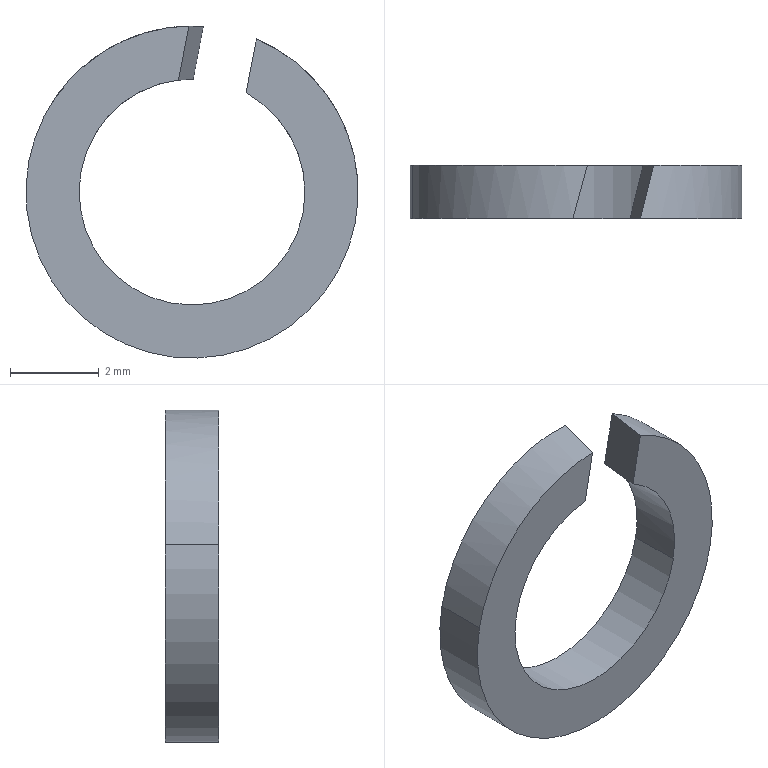Component | SolidWorks | SpringWasher_5-2 | 1 solid | 10 faces | box 7.5 x 1.2 x 7.5 mm | volume 26 mm3 | cylinder 6 | plane 4 | commonest cylinder face diameters 5.1 x3 7.5 x3 | material Plain Carbon Steel
build123d program:
from build123d import *

# Parameters (mm, degrees)
SKETCH1_R           = 3.75
SKETCH1_R_2         = 2.55
BOSS_EXTRUDE1_DEPTH = 1.2
CUT_EXTRUDE1_DEPTH  = 6.437


with BuildPart() as part:
    # Sketch1 → Boss-Extrude1 (new body)
    with BuildSketch(Plane.XY):
        Circle(SKETCH1_R)
        Circle(SKETCH1_R_2, mode=Mode.SUBTRACT)
    extrude(amount=BOSS_EXTRUDE1_DEPTH)

    # Sketch2 → Cut-Extrude1 (cut, through all)
    with BuildSketch(Plane(origin=(0, 0, 0), x_dir=(1, 0, 0), z_dir=(0, 1, 0))):
        Polygon((-0.4549, -1.2), (-0.7765, 0), (0.7765, 0), (1.098, -1.2), align=None)
    extrude(amount=-CUT_EXTRUDE1_DEPTH, mode=Mode.SUBTRACT)


solid = part.part

# Placed as in the assembly
solid = solid.moved(Location((-144.749, -17, 133.251), (-90, 0, 10.863)))
STEP:
#1=CARTESIAN_POINT('',(-5.639,-0.622,5.327));
#2=VERTEX_POINT('',#1);
#3=CARTESIAN_POINT('',(-5.6,-0.622,5.227));
#4=VERTEX_POINT('',#3);
#5=CARTESIAN_POINT('',(-5.699,-0.622,5.246));
#6=DIRECTION('',(-0.,1.,0.));
#7=DIRECTION('',(0.9821,0.,-0.1885));
#8=AXIS2_PLACEMENT_3D('',#5,#6,#7);
#9=CIRCLE('',#8,0.1004);
#10=EDGE_CURVE('',#2,#4,#9,.T.);
#11=ORIENTED_EDGE('',*,*,#10,.T.);
#12=CARTESIAN_POINT('',(-5.6,-0.6693,5.227));
#13=VERTEX_POINT('',#12);
#14=CARTESIAN_POINT('',(-5.6,-0.622,5.227));
#15=DIRECTION('',(0.,-1.,-0.));
#16=VECTOR('',#15,39.37);
#17=LINE('',#14,#16);
#18=EDGE_CURVE('',#4,#13,#17,.T.);
#19=ORIENTED_EDGE('',*,*,#18,.T.);
#20=CARTESIAN_POINT('',(-5.651,-0.6693,5.334));
#21=VERTEX_POINT('',#20);
#22=CARTESIAN_POINT('',(-5.699,-0.6693,5.246));
#23=DIRECTION('',(-0.,1.,0.));
#24=DIRECTION('',(0.9821,0.,-0.1885));
#25=AXIS2_PLACEMENT_3D('',#22,#23,#24);
#26=CIRCLE('',#25,0.1004);
#27=EDGE_CURVE('',#21,#13,#26,.T.);
#28=ORIENTED_EDGE('',*,*,#27,.F.);
#29=CARTESIAN_POINT('',(-5.639,-0.622,5.327));
#30=CARTESIAN_POINT('',(-5.643,-0.6374,5.33));
#31=CARTESIAN_POINT('',(-5.647,-0.6531,5.332));
#32=CARTESIAN_POINT('',(-5.651,-0.6693,5.334));
#33=(BOUNDED_CURVE()B_SPLINE_CURVE(3,(#29,#30,#31,#32),.UNSPECIFIED.,.F.,.F.)B_SPLINE_CURVE_WITH_KNOTS((4,4),(4.267,4.403),.UNSPECIFIED.)CURVE()GEOMETRIC_REPRESENTATION_ITEM()RATIONAL_B_SPLINE_CURVE((1.,0.9985,0.9985,1.))REPRESENTATION_ITEM(''));
#34=EDGE_CURVE('',#2,#21,#33,.T.);
#35=ORIENTED_EDGE('',*,*,#34,.F.);
#36=EDGE_LOOP('',(#11,#19,#28,#35));
#37=FACE_OUTER_BOUND('',#36,.T.);
#38=CARTESIAN_POINT('',(-5.699,-0.622,5.246));
#39=DIRECTION('',(0.,-1.,-0.));
#40=DIRECTION('',(-0.9821,0.,0.1885));
#41=AXIS2_PLACEMENT_3D('',#38,#39,#40);
#42=CYLINDRICAL_SURFACE('',#41,0.1004);
#43=ADVANCED_FACE('',(#37),#42,.F.);
#44=ORIENTED_EDGE('',*,*,#18,.F.);
#45=CARTESIAN_POINT('',(-5.797,-0.622,5.265));
#46=VERTEX_POINT('',#45);
#47=CARTESIAN_POINT('',(-5.699,-0.622,5.246));
#48=DIRECTION('',(-0.,1.,0.));
#49=DIRECTION('',(0.9821,0.,-0.1885));
#50=AXIS2_PLACEMENT_3D('',#47,#48,#49);
#51=CIRCLE('',#50,0.1004);
#52=EDGE_CURVE('',#4,#46,#51,.T.);
#53=ORIENTED_EDGE('',*,*,#52,.T.);
#54=CARTESIAN_POINT('',(-5.797,-0.6693,5.265));
#55=VERTEX_POINT('',#54);
#56=CARTESIAN_POINT('',(-5.797,-0.622,5.265));
#57=DIRECTION('',(0.,-1.,-0.));
#58=VECTOR('',#57,39.37);
#59=LINE('',#56,#58);
#60=EDGE_CURVE('',#46,#55,#59,.T.);
#61=ORIENTED_EDGE('',*,*,#60,.T.);
#62=CARTESIAN_POINT('',(-5.699,-0.6693,5.246));
#63=DIRECTION('',(-0.,1.,0.));
#64=DIRECTION('',(0.9821,0.,-0.1885));
#65=AXIS2_PLACEMENT_3D('',#62,#63,#64);
#66=CIRCLE('',#65,0.1004);
#67=EDGE_CURVE('',#13,#55,#66,.T.);
#68=ORIENTED_EDGE('',*,*,#67,.F.);
#69=EDGE_LOOP('',(#44,#53,#61,#68));
#70=FACE_OUTER_BOUND('',#69,.T.);
#71=CARTESIAN_POINT('',(-5.699,-0.622,5.246));
#72=DIRECTION('',(0.,-1.,-0.));
#73=DIRECTION('',(-0.9821,0.,0.1885));
#74=AXIS2_PLACEMENT_3D('',#71,#72,#73);
#75=CYLINDRICAL_SURFACE('',#74,0.1004);
#76=ADVANCED_FACE('',(#70),#75,.F.);
#77=CARTESIAN_POINT('',(-5.554,-0.622,5.218));
#78=VERTEX_POINT('',#77);
#79=CARTESIAN_POINT('',(-5.844,-0.622,5.274));
#80=VERTEX_POINT('',#79);
#81=CARTESIAN_POINT('',(-5.699,-0.622,5.246));
#82=DIRECTION('',(-0.,1.,0.));
#83=DIRECTION('',(0.9821,0.,-0.1885));
#84=AXIS2_PLACEMENT_3D('',#81,#82,#83);
#85=CIRCLE('',#84,0.1476);
#86=EDGE_CURVE('',#78,#80,#85,.T.);
#87=ORIENTED_EDGE('',*,*,#86,.F.);
#88=CARTESIAN_POINT('',(-5.554,-0.6693,5.218));
#89=VERTEX_POINT('',#88);
#90=CARTESIAN_POINT('',(-5.554,-0.622,5.218));
#91=DIRECTION('',(0.,-1.,-0.));
#92=VECTOR('',#91,39.37);
#93=LINE('',#90,#92);
#94=EDGE_CURVE('',#78,#89,#93,.T.);
#95=ORIENTED_EDGE('',*,*,#94,.T.);
#96=CARTESIAN_POINT('',(-5.844,-0.6693,5.274));
#97=VERTEX_POINT('',#96);
#98=CARTESIAN_POINT('',(-5.699,-0.6693,5.246));
#99=DIRECTION('',(-0.,1.,0.));
#100=DIRECTION('',(0.9821,0.,-0.1885));
#101=AXIS2_PLACEMENT_3D('',#98,#99,#100);
#102=CIRCLE('',#101,0.1476);
#103=EDGE_CURVE('',#89,#97,#102,.T.);
#104=ORIENTED_EDGE('',*,*,#103,.T.);
#105=CARTESIAN_POINT('',(-5.844,-0.622,5.274));
#106=DIRECTION('',(0.,-1.,-0.));
#107=VECTOR('',#106,39.37);
#108=LINE('',#105,#107);
#109=EDGE_CURVE('',#80,#97,#108,.T.);
#110=ORIENTED_EDGE('',*,*,#109,.F.);
#111=EDGE_LOOP('',(#87,#95,#104,#110));
#112=FACE_OUTER_BOUND('',#111,.T.);
#113=CARTESIAN_POINT('',(-5.699,-0.622,5.246));
#114=DIRECTION('',(0.,-1.,-0.));
#115=DIRECTION('',(-0.9821,0.,0.1885));
#116=AXIS2_PLACEMENT_3D('',#113,#114,#115);
#117=CYLINDRICAL_SURFACE('',#116,0.1476);
#118=ADVANCED_FACE('',(#112),#117,.T.);
#119=CARTESIAN_POINT('',(-5.689,-0.622,5.393));
#120=VERTEX_POINT('',#119);
#121=CARTESIAN_POINT('',(-5.699,-0.622,5.246));
#122=DIRECTION('',(-0.,1.,0.));
#123=DIRECTION('',(0.9821,0.,-0.1885));
#124=AXIS2_PLACEMENT_3D('',#121,#122,#123);
#125=CIRCLE('',#124,0.1476);
#126=EDGE_CURVE('',#80,#120,#125,.T.);
#127=ORIENTED_EDGE('',*,*,#126,.F.);
#128=ORIENTED_EDGE('',*,*,#109,.T.);
#129=CARTESIAN_POINT('',(-5.702,-0.6693,5.394));
#130=VERTEX_POINT('',#129);
#131=CARTESIAN_POINT('',(-5.699,-0.6693,5.246));
#132=DIRECTION('',(-0.,1.,0.));
#133=DIRECTION('',(0.9821,0.,-0.1885));
#134=AXIS2_PLACEMENT_3D('',#131,#132,#133);
#135=CIRCLE('',#134,0.1476);
#136=EDGE_CURVE('',#97,#130,#135,.T.);
#137=ORIENTED_EDGE('',*,*,#136,.T.);
#138=CARTESIAN_POINT('',(-5.702,-0.6693,5.394));
#139=CARTESIAN_POINT('',(-5.697,-0.6537,5.394));
#140=CARTESIAN_POINT('',(-5.693,-0.6379,5.394));
#141=CARTESIAN_POINT('',(-5.689,-0.622,5.393));
#142=(BOUNDED_CURVE()B_SPLINE_CURVE(3,(#138,#139,#140,#141),.UNSPECIFIED.,.F.,.T.)B_SPLINE_CURVE_WITH_KNOTS((4,4),(1.362,1.449),.UNSPECIFIED.)CURVE()GEOMETRIC_REPRESENTATION_ITEM()RATIONAL_B_SPLINE_CURVE((1.,0.9994,0.9994,1.))REPRESENTATION_ITEM(''));
#143=EDGE_CURVE('',#130,#120,#142,.T.);
#144=ORIENTED_EDGE('',*,*,#143,.T.);
#145=EDGE_LOOP('',(#127,#128,#137,#144));
#146=FACE_OUTER_BOUND('',#145,.T.);
#147=CARTESIAN_POINT('',(-5.699,-0.622,5.246));
#148=DIRECTION('',(0.,-1.,-0.));
#149=DIRECTION('',(-0.9821,0.,0.1885));
#150=AXIS2_PLACEMENT_3D('',#147,#148,#149);
#151=CYLINDRICAL_SURFACE('',#150,0.1476);
#152=ADVANCED_FACE('',(#146),#151,.T.);
#153=CARTESIAN_POINT('',(-5.698,-0.622,5.347));
#154=VERTEX_POINT('',#153);
#155=CARTESIAN_POINT('',(-5.689,-0.622,5.394));
#156=DIRECTION('',(-0.1885,0.,-0.9821));
#157=VECTOR('',#156,39.37);
#158=LINE('',#155,#157);
#159=EDGE_CURVE('',#120,#154,#158,.T.);
#160=ORIENTED_EDGE('',*,*,#159,.T.);
#161=CARTESIAN_POINT('',(-5.699,-0.622,5.246));
#162=DIRECTION('',(-0.,1.,0.));
#163=DIRECTION('',(0.9821,0.,-0.1885));
#164=AXIS2_PLACEMENT_3D('',#161,#162,#163);
#165=CIRCLE('',#164,0.1004);
#166=EDGE_CURVE('',#46,#154,#165,.T.);
#167=ORIENTED_EDGE('',*,*,#166,.F.);
#168=ORIENTED_EDGE('',*,*,#52,.F.);
#169=ORIENTED_EDGE('',*,*,#10,.F.);
#170=CARTESIAN_POINT('',(-5.63,-0.622,5.377));
#171=VERTEX_POINT('',#170);
#172=CARTESIAN_POINT('',(-5.628,-0.622,5.383));
#173=DIRECTION('',(-0.1885,0.,-0.9821));
#174=VECTOR('',#173,39.37);
#175=LINE('',#172,#174);
#176=EDGE_CURVE('',#171,#2,#175,.T.);
#177=ORIENTED_EDGE('',*,*,#176,.F.);
#178=CARTESIAN_POINT('',(-5.699,-0.622,5.246));
#179=DIRECTION('',(-0.,1.,0.));
#180=DIRECTION('',(0.9821,0.,-0.1885));
#181=AXIS2_PLACEMENT_3D('',#178,#179,#180);
#182=CIRCLE('',#181,0.1476);
#183=EDGE_CURVE('',#171,#78,#182,.T.);
#184=ORIENTED_EDGE('',*,*,#183,.T.);
#185=ORIENTED_EDGE('',*,*,#86,.T.);
#186=ORIENTED_EDGE('',*,*,#126,.T.);
#187=EDGE_LOOP('',(#160,#167,#168,#169,#177,#184,#185,#186));
#188=FACE_OUTER_BOUND('',#187,.T.);
#189=CARTESIAN_POINT('',(-5.699,-0.622,5.246));
#190=DIRECTION('',(-0.,1.,0.));
#191=DIRECTION('',(0.9821,0.,-0.1885));
#192=AXIS2_PLACEMENT_3D('',#189,#190,#191);
#193=PLANE('',#192);
#194=ADVANCED_FACE('',(#188),#193,.T.);
#195=ORIENTED_EDGE('',*,*,#27,.T.);
#196=ORIENTED_EDGE('',*,*,#67,.T.);
#197=CARTESIAN_POINT('',(-5.711,-0.6693,5.346));
#198=VERTEX_POINT('',#197);
#199=CARTESIAN_POINT('',(-5.699,-0.6693,5.246));
#200=DIRECTION('',(-0.,1.,0.));
#201=DIRECTION('',(0.9821,0.,-0.1885));
#202=AXIS2_PLACEMENT_3D('',#199,#200,#201);
#203=CIRCLE('',#202,0.1004);
#204=EDGE_CURVE('',#55,#198,#203,.T.);
#205=ORIENTED_EDGE('',*,*,#204,.T.);
#206=CARTESIAN_POINT('',(-5.701,-0.6693,5.397));
#207=DIRECTION('',(-0.1885,0.,-0.9821));
#208=VECTOR('',#207,39.37);
#209=LINE('',#206,#208);
#210=EDGE_CURVE('',#130,#198,#209,.T.);
#211=ORIENTED_EDGE('',*,*,#210,.F.);
#212=ORIENTED_EDGE('',*,*,#136,.F.);
#213=ORIENTED_EDGE('',*,*,#103,.F.);
#214=CARTESIAN_POINT('',(-5.642,-0.6693,5.382));
#215=VERTEX_POINT('',#214);
#216=CARTESIAN_POINT('',(-5.699,-0.6693,5.246));
#217=DIRECTION('',(-0.,1.,0.));
#218=DIRECTION('',(0.9821,0.,-0.1885));
#219=AXIS2_PLACEMENT_3D('',#216,#217,#218);
#220=CIRCLE('',#219,0.1476);
#221=EDGE_CURVE('',#215,#89,#220,.T.);
#222=ORIENTED_EDGE('',*,*,#221,.F.);
#223=CARTESIAN_POINT('',(-5.641,-0.6693,5.385));
#224=DIRECTION('',(-0.1885,0.,-0.9821));
#225=VECTOR('',#224,39.37);
#226=LINE('',#223,#225);
#227=EDGE_CURVE('',#215,#21,#226,.T.);
#228=ORIENTED_EDGE('',*,*,#227,.T.);
#229=EDGE_LOOP('',(#195,#196,#205,#211,#212,#213,#222,#228));
#230=FACE_OUTER_BOUND('',#229,.T.);
#231=CARTESIAN_POINT('',(-5.699,-0.6693,5.246));
#232=DIRECTION('',(-0.,1.,0.));
#233=DIRECTION('',(0.9821,0.,-0.1885));
#234=AXIS2_PLACEMENT_3D('',#231,#232,#233);
#235=PLANE('',#234);
#236=ADVANCED_FACE('',(#230),#235,.F.);
#237=ORIENTED_EDGE('',*,*,#94,.F.);
#238=ORIENTED_EDGE('',*,*,#183,.F.);
#239=CARTESIAN_POINT('',(-5.63,-0.622,5.377));
#240=CARTESIAN_POINT('',(-5.634,-0.6376,5.379));
#241=CARTESIAN_POINT('',(-5.638,-0.6534,5.381));
#242=CARTESIAN_POINT('',(-5.642,-0.6693,5.382));
#243=(BOUNDED_CURVE()B_SPLINE_CURVE(3,(#239,#240,#241,#242),.UNSPECIFIED.,.F.,.F.)B_SPLINE_CURVE_WITH_KNOTS((4,4),(4.415,4.504),.UNSPECIFIED.)CURVE()GEOMETRIC_REPRESENTATION_ITEM()RATIONAL_B_SPLINE_CURVE((1.,0.9993,0.9993,1.))REPRESENTATION_ITEM(''));
#244=EDGE_CURVE('',#171,#215,#243,.T.);
#245=ORIENTED_EDGE('',*,*,#244,.T.);
#246=ORIENTED_EDGE('',*,*,#221,.T.);
#247=EDGE_LOOP('',(#237,#238,#245,#246));
#248=FACE_OUTER_BOUND('',#247,.T.);
#249=CARTESIAN_POINT('',(-5.699,-0.622,5.246));
#250=DIRECTION('',(0.,-1.,-0.));
#251=DIRECTION('',(-0.9821,0.,0.1885));
#252=AXIS2_PLACEMENT_3D('',#249,#250,#251);
#253=CYLINDRICAL_SURFACE('',#252,0.1476);
#254=ADVANCED_FACE('',(#248),#253,.T.);
#255=ORIENTED_EDGE('',*,*,#60,.F.);
#256=ORIENTED_EDGE('',*,*,#166,.T.);
#257=CARTESIAN_POINT('',(-5.711,-0.6693,5.346));
#258=CARTESIAN_POINT('',(-5.706,-0.6538,5.346));
#259=CARTESIAN_POINT('',(-5.702,-0.638,5.347));
#260=CARTESIAN_POINT('',(-5.698,-0.622,5.347));
#261=(BOUNDED_CURVE()B_SPLINE_CURVE(3,(#257,#258,#259,#260),.UNSPECIFIED.,.F.,.T.)B_SPLINE_CURVE_WITH_KNOTS((4,4),(1.261,1.391),.UNSPECIFIED.)CURVE()GEOMETRIC_REPRESENTATION_ITEM()RATIONAL_B_SPLINE_CURVE((1.,0.9986,0.9986,1.))REPRESENTATION_ITEM(''));
#262=EDGE_CURVE('',#198,#154,#261,.T.);
#263=ORIENTED_EDGE('',*,*,#262,.F.);
#264=ORIENTED_EDGE('',*,*,#204,.F.);
#265=EDGE_LOOP('',(#255,#256,#263,#264));
#266=FACE_OUTER_BOUND('',#265,.T.);
#267=CARTESIAN_POINT('',(-5.699,-0.622,5.246));
#268=DIRECTION('',(0.,-1.,-0.));
#269=DIRECTION('',(-0.9821,0.,0.1885));
#270=AXIS2_PLACEMENT_3D('',#267,#268,#269);
#271=CYLINDRICAL_SURFACE('',#270,0.1004);
#272=ADVANCED_FACE('',(#266),#271,.F.);
#273=ORIENTED_EDGE('',*,*,#176,.T.);
#274=ORIENTED_EDGE('',*,*,#34,.T.);
#275=ORIENTED_EDGE('',*,*,#227,.F.);
#276=ORIENTED_EDGE('',*,*,#244,.F.);
#277=EDGE_LOOP('',(#273,#274,#275,#276));
#278=FACE_OUTER_BOUND('',#277,.T.);
#279=CARTESIAN_POINT('',(-5.641,-0.6693,5.385));
#280=DIRECTION('',(0.9486,-0.2588,-0.182));
#281=DIRECTION('',(-0.2542,-0.9659,0.04878));
#282=AXIS2_PLACEMENT_3D('',#279,#280,#281);
#283=PLANE('',#282);
#284=ADVANCED_FACE('',(#278),#283,.F.);
#285=ORIENTED_EDGE('',*,*,#210,.T.);
#286=ORIENTED_EDGE('',*,*,#262,.T.);
#287=ORIENTED_EDGE('',*,*,#159,.F.);
#288=ORIENTED_EDGE('',*,*,#143,.F.);
#289=EDGE_LOOP('',(#285,#286,#287,#288));
#290=FACE_OUTER_BOUND('',#289,.T.);
#291=CARTESIAN_POINT('',(-5.689,-0.622,5.394));
#292=DIRECTION('',(-0.9486,0.2588,0.182));
#293=DIRECTION('',(0.2542,0.9659,-0.04878));
#294=AXIS2_PLACEMENT_3D('',#291,#292,#293);
#295=PLANE('',#294);
#296=ADVANCED_FACE('',(#290),#295,.F.);
#297=CLOSED_SHELL('',(#43,#76,#118,#152,#194,#236,#254,#272,#284,#296));
#298=MANIFOLD_SOLID_BREP('',#297);
#299=CARTESIAN_POINT('',(0.,0.,0.));
#300=DIRECTION('',(0.,0.,1.));
#301=DIRECTION('',(1.,0.,0.));
#302=AXIS2_PLACEMENT_3D('',#299,#300,#301);
#303=(LENGTH_UNIT()NAMED_UNIT(*)SI_UNIT($,.METRE.));
#304=LENGTH_MEASURE_WITH_UNIT(LENGTH_MEASURE(0.0254),#303);
#305=DIMENSIONAL_EXPONENTS(1.,0.,0.,0.,0.,0.,0.);
#306=(CONVERSION_BASED_UNIT('',#304)LENGTH_UNIT()NAMED_UNIT(#305));
#307=UNCERTAINTY_MEASURE_WITH_UNIT(LENGTH_MEASURE(0.00001),#306,'','');
#308=(NAMED_UNIT(*)PLANE_ANGLE_UNIT()SI_UNIT($,.RADIAN.));
#309=(NAMED_UNIT(*)SI_UNIT($,.STERADIAN.)SOLID_ANGLE_UNIT());
#310=(GEOMETRIC_REPRESENTATION_CONTEXT(3)GLOBAL_UNCERTAINTY_ASSIGNED_CONTEXT((#307))GLOBAL_UNIT_ASSIGNED_CONTEXT((#306,#308,#309))REPRESENTATION_CONTEXT('',''));
#311=ADVANCED_BREP_SHAPE_REPRESENTATION('',(#298,#302),#310);
#312=COLOUR_RGB('',0.7922,0.8196,0.9333);
#313=FILL_AREA_STYLE_COLOUR('',#312);
#314=FILL_AREA_STYLE('',(#313));
#315=SURFACE_STYLE_FILL_AREA(#314);
#316=SURFACE_SIDE_STYLE('',(#315));
#317=SURFACE_STYLE_USAGE(.BOTH.,#316);
#318=PRESENTATION_STYLE_ASSIGNMENT((#317));
#319=STYLED_ITEM('',(#318),#298);
#320=(LENGTH_UNIT()NAMED_UNIT(*)SI_UNIT($,.METRE.));
#321=LENGTH_MEASURE_WITH_UNIT(LENGTH_MEASURE(0.0254),#320);
#322=DIMENSIONAL_EXPONENTS(1.,0.,0.,0.,0.,0.,0.);
#323=(CONVERSION_BASED_UNIT('',#321)LENGTH_UNIT()NAMED_UNIT(#322));
#324=UNCERTAINTY_MEASURE_WITH_UNIT(LENGTH_MEASURE(0.00001),#323,'','');
#325=(NAMED_UNIT(*)PLANE_ANGLE_UNIT()SI_UNIT($,.RADIAN.));
#326=(NAMED_UNIT(*)SI_UNIT($,.STERADIAN.)SOLID_ANGLE_UNIT());
#327=(GEOMETRIC_REPRESENTATION_CONTEXT(3)GLOBAL_UNCERTAINTY_ASSIGNED_CONTEXT((#324))GLOBAL_UNIT_ASSIGNED_CONTEXT((#323,#325,#326))REPRESENTATION_CONTEXT('',''));
#328=MECHANICAL_DESIGN_GEOMETRIC_PRESENTATION_REPRESENTATION('',(#319),#327);
#329=PRESENTATION_LAYER_ASSIGNMENT('','',(#319));